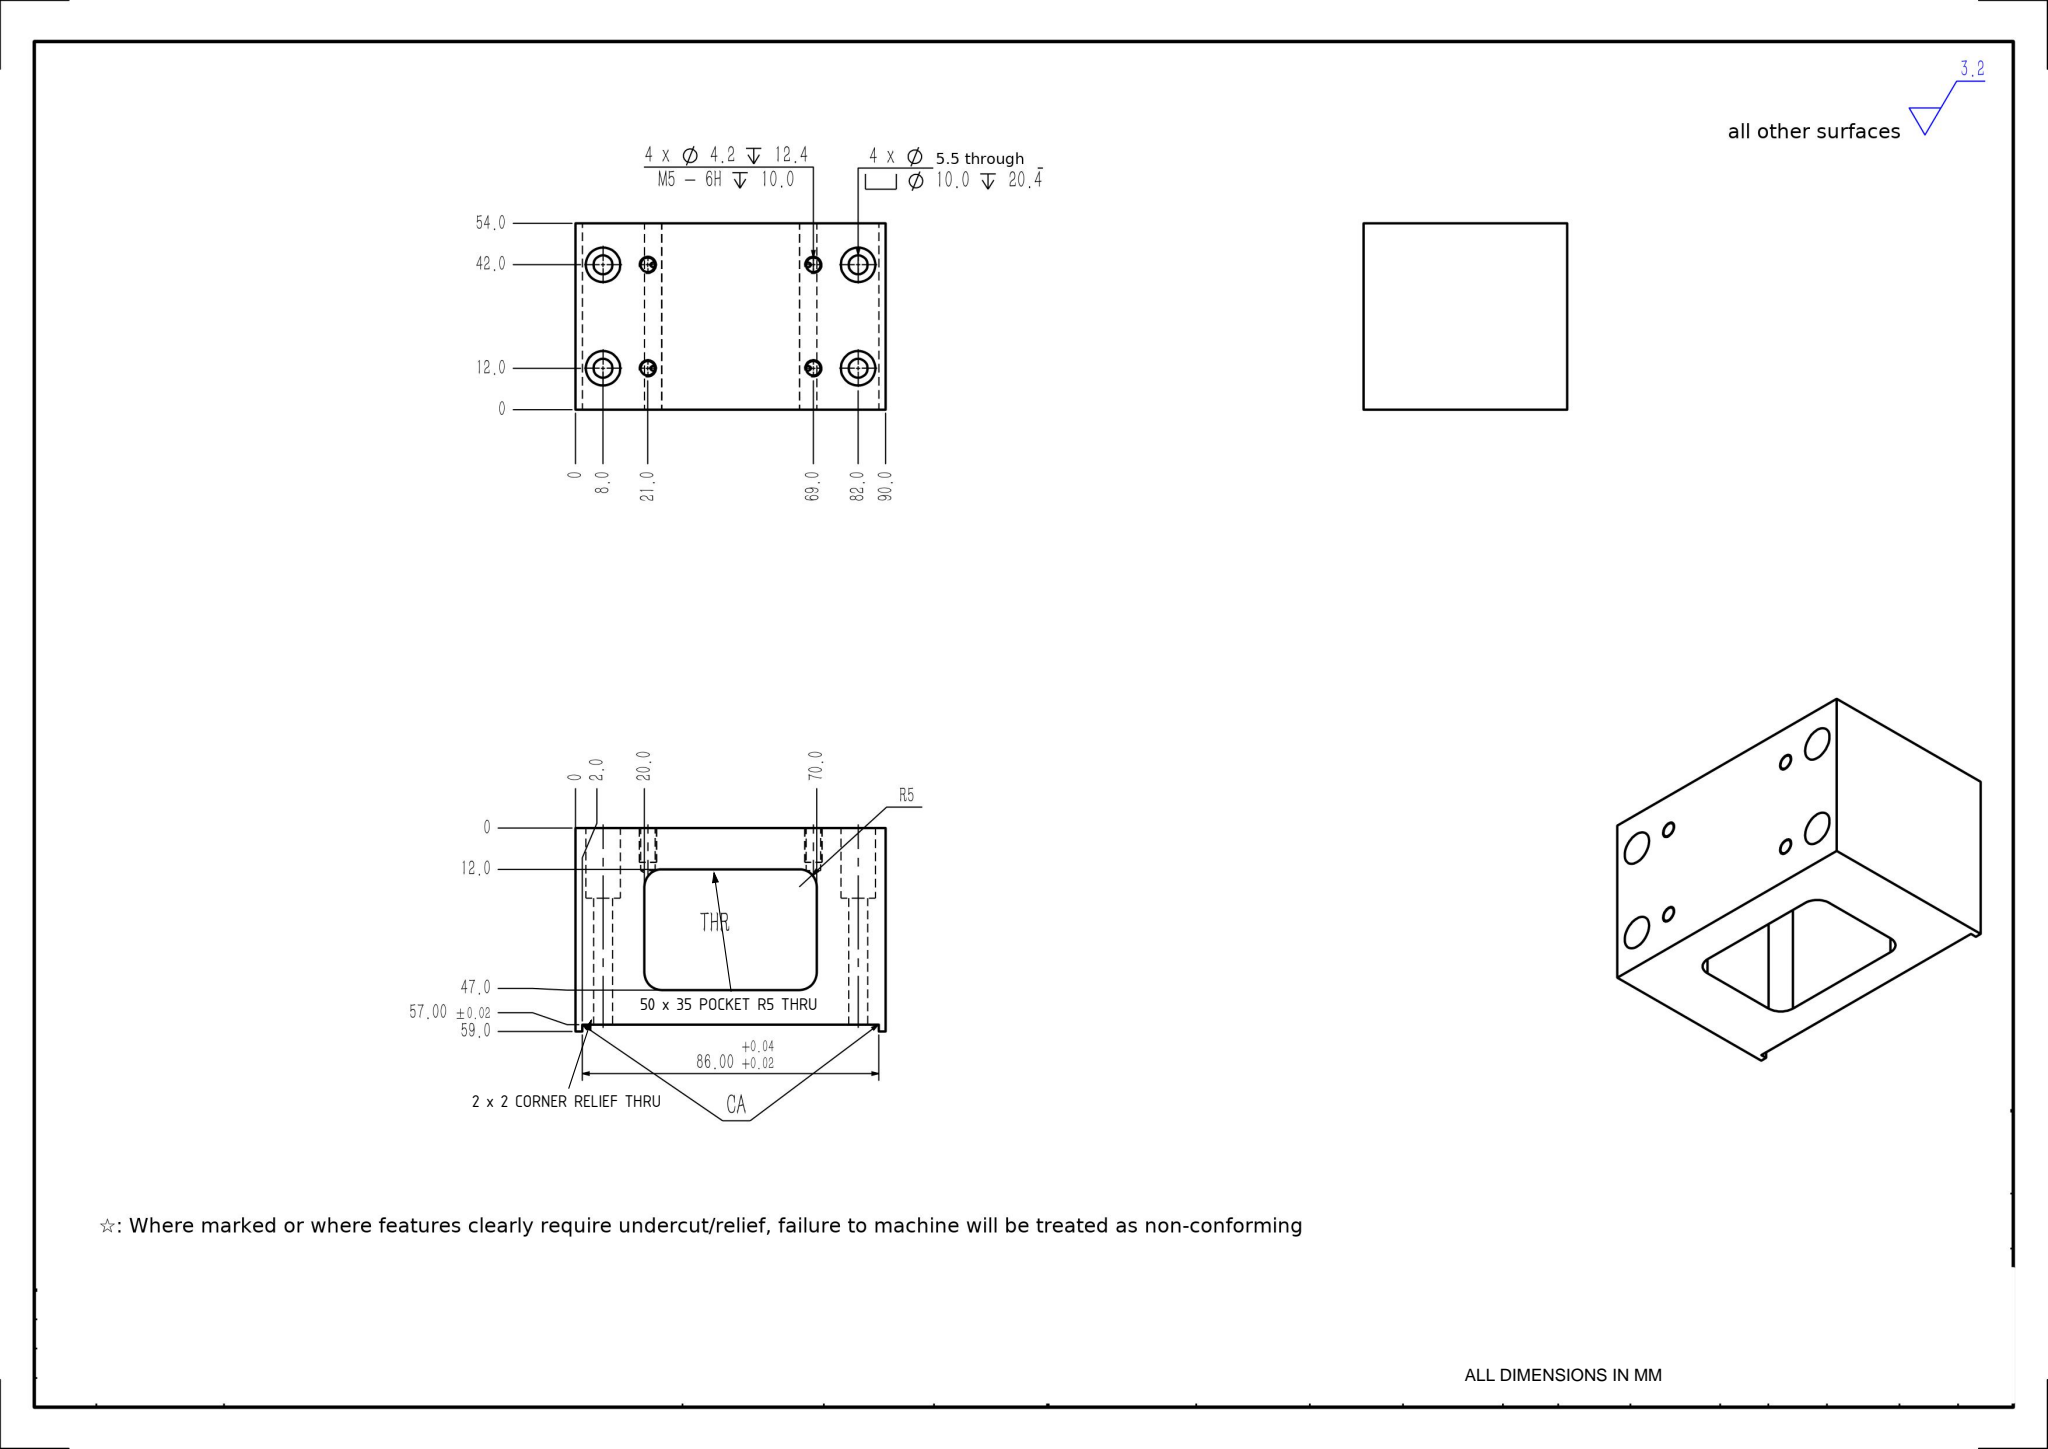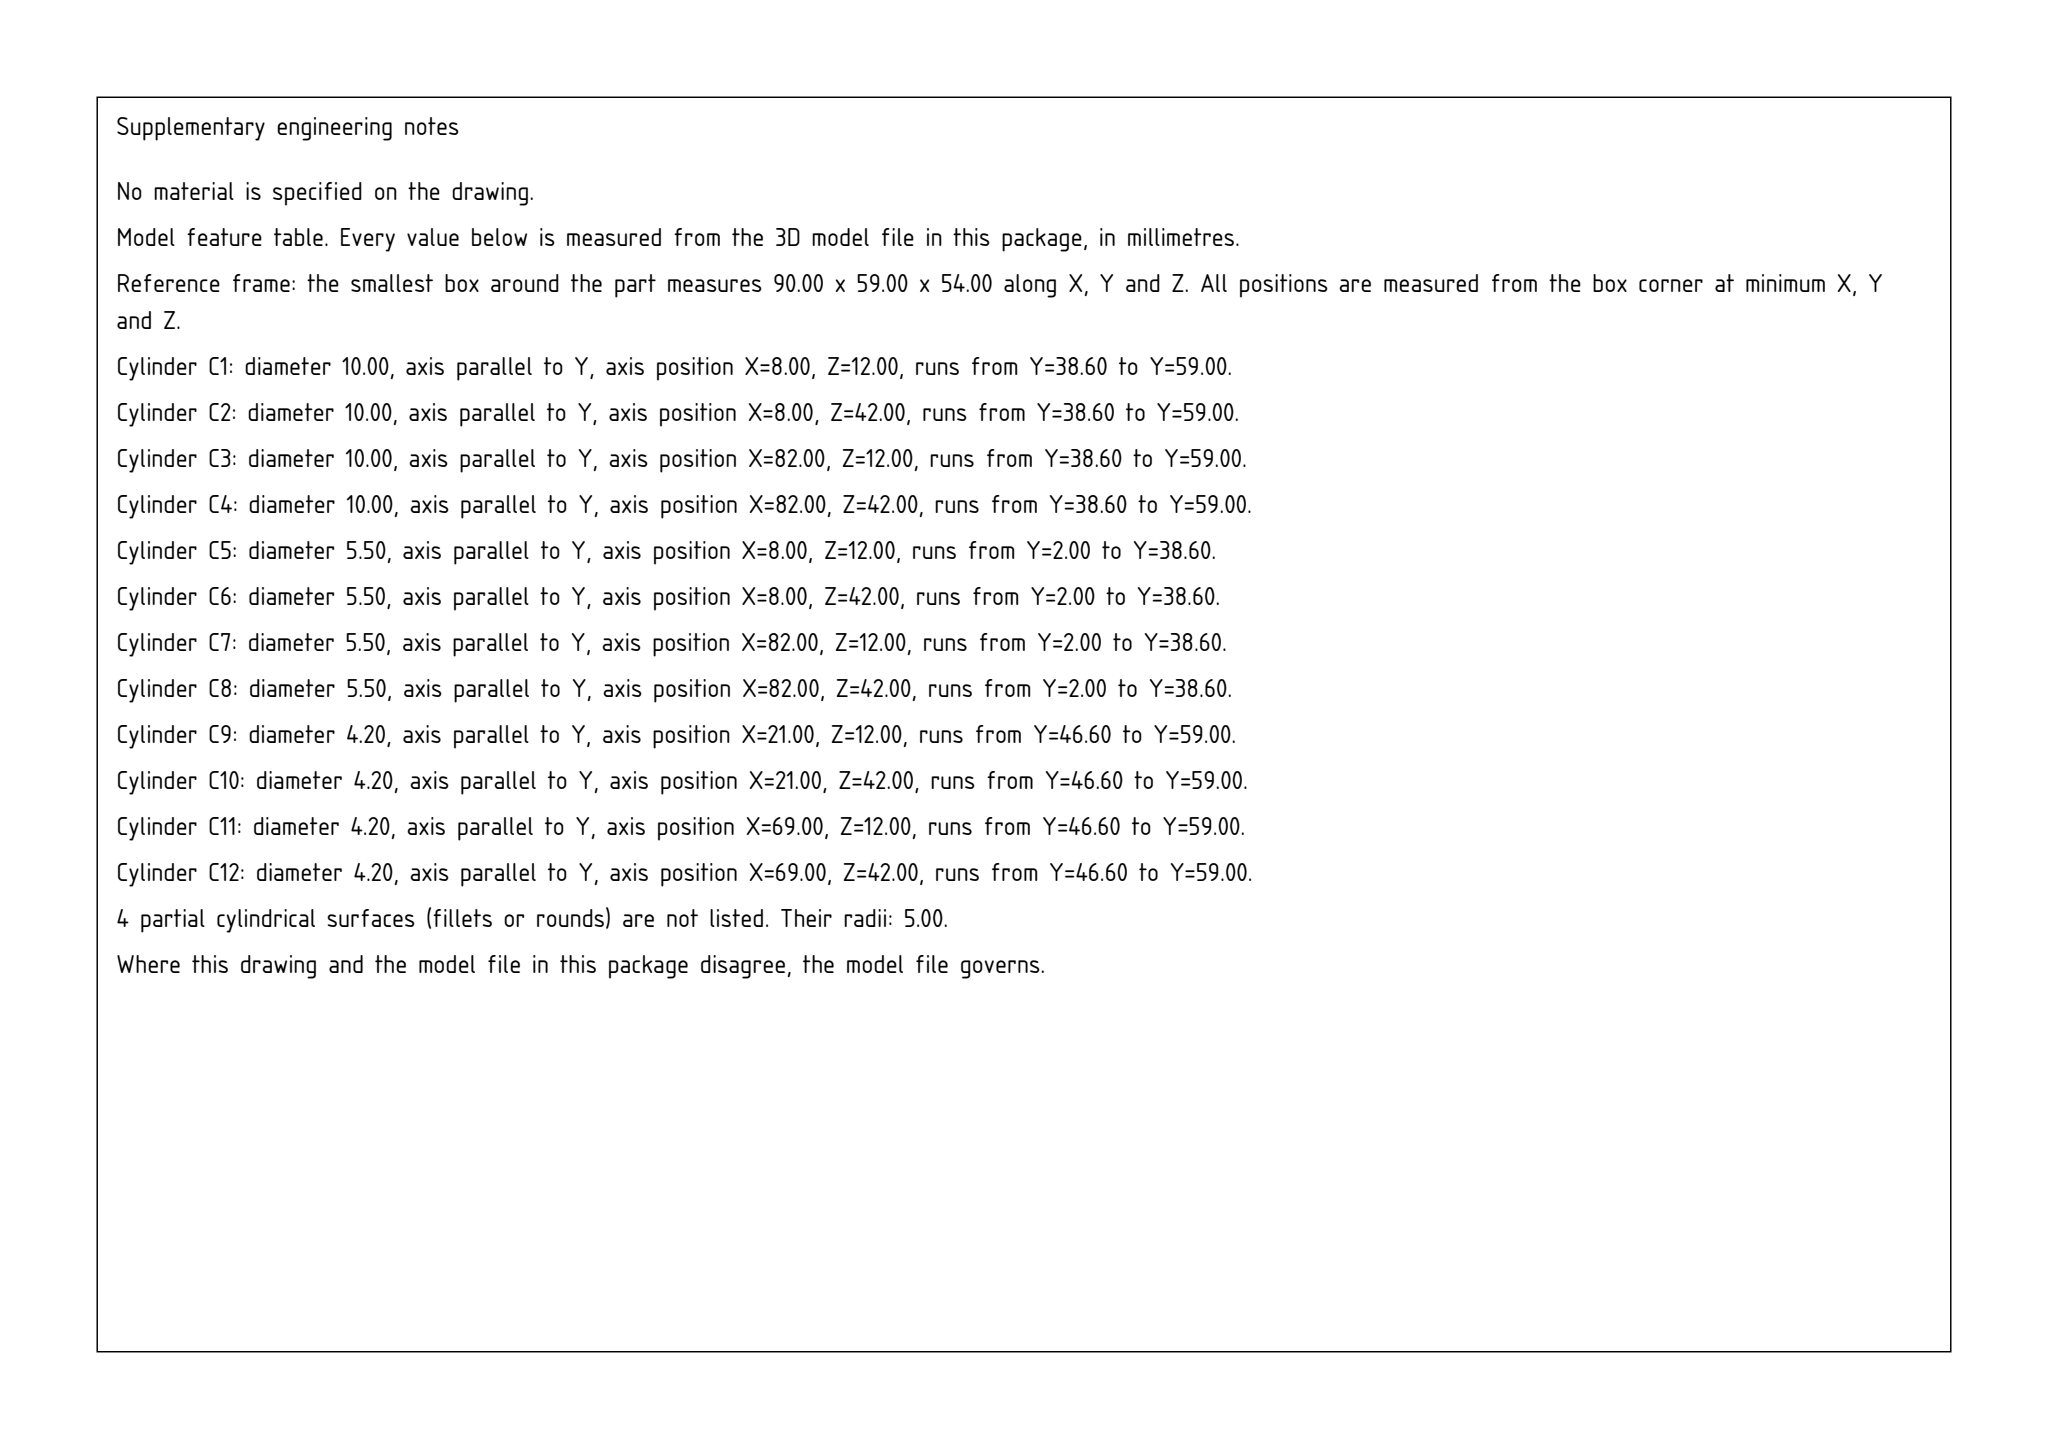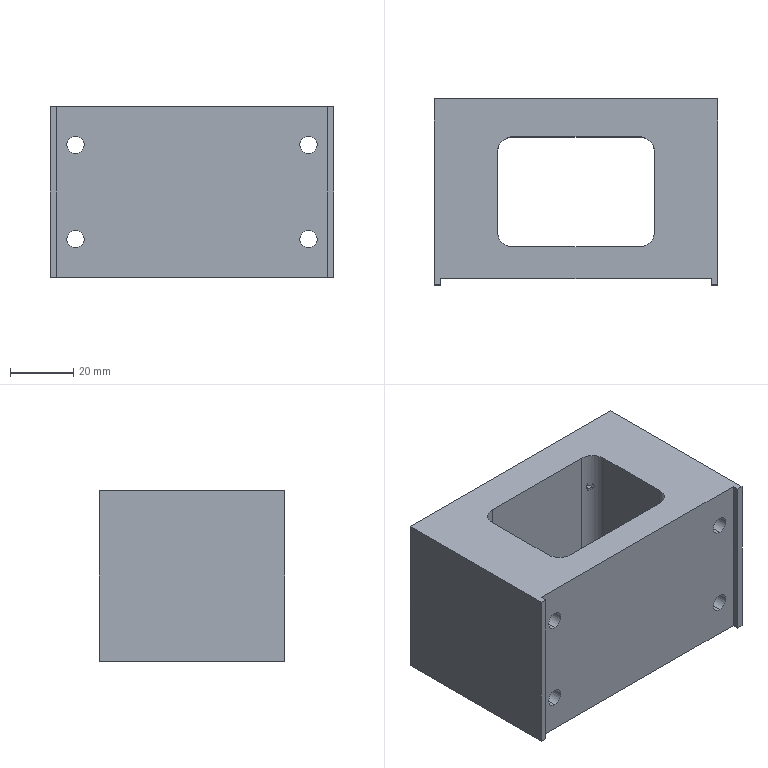Part | SolidWorks | mm | 1 solid | 54 faces | box 90 x 59 x 54 mm | volume 173514 mm3 | cylinder 28 | plane 18 | cone 8 | commonest cylinder face diameters 10 x12 4.2 x8 5.5 x8
Drawing notes:
RECT POCKET 50 x 35, R5 CORNERS, THRU | from the solid: Pocket faces x=20 & x=70 (50 wide), y=12 & y=47 (35 high); four R5 corner cyls Ø10 axis z at (25,17),(25,42),(65,17),(65,42) length 54 = full block depth, i.e. thru
CORNER RELIEF 2 x 2, BOTH BOT CORNERS, THRU 54 DEPTH | from the solid: Planes x=2.0 & x=88.0 (86.00 across) with plane y=2.0 (57.00 from top face y=59) vs bbox 90 x 59 x 54; relief runs full 54 depth
build123d program:
from build123d import *

# Parameters (mm, degrees)
BOSS_EXTRUDE1_DEPTH                             = 27
CUT_EXTRUDE1_DEPTH                              = 77.232
M5_HEX_SOCKET_HEAD_CAP_SCREW_CBORE1_D           = 5.5
M5_HEX_SOCKET_HEAD_CAP_SCREW_CBORE1_CBORE_D     = 10
M5_HEX_SOCKET_HEAD_CAP_SCREW_CBORE1_CBORE_DEPTH = 20.4
M5_TAPPED_HOLE1_D                               = 4.2
M5_TAPPED_HOLE1_DEPTH                           = 12.4
M5_TAPPED_HOLE1_TIP                             = 1.262


with BuildPart() as part:
    # Sketch1 → Boss-Extrude1 (new, symmetric)
    with BuildSketch(Plane.XY):
        Polygon((-43, -29.5), (-43, -27.5), (43, -27.5), (43, -29.5), (45, -29.5), (45, 29.5), (-45, 29.5), (-45, -29.5), align=None)
    extrude(amount=BOSS_EXTRUDE1_DEPTH, both=True)

    # Sketch2 → Cut-Extrude1 (cut, through all)
    with BuildSketch(Plane.XY.offset(27)):
        with BuildLine():
            Line((-20, -17.5), (20, -17.5))
            ThreePointArc((20, -17.5), (23.536, -16.036), (25, -12.5))
            Line((25, -12.5), (25, 12.5))
            ThreePointArc((25, 12.5), (23.536, 16.036), (20, 17.5))
            Line((20, 17.5), (-20, 17.5))
            ThreePointArc((-20, 17.5), (-23.536, 16.036), (-25, 12.5))
            Line((-25, 12.5), (-25, -12.5))
            ThreePointArc((-25, -12.5), (-23.536, -16.036), (-20, -17.5))
        make_face()
    extrude(amount=-CUT_EXTRUDE1_DEPTH, mode=Mode.SUBTRACT)

    # M5 Hex Socket Head Cap Screw CBORE1 (through all)
    with Locations(Plane(origin=(0, 29.5, 0), x_dir=(1, 0, 0), z_dir=(0, 1, 0))):
        with Locations((-37, 15), (-37, -15), (37, 15), (37, -15)):
            CounterBoreHole(M5_HEX_SOCKET_HEAD_CAP_SCREW_CBORE1_D / 2, M5_HEX_SOCKET_HEAD_CAP_SCREW_CBORE1_CBORE_D / 2, M5_HEX_SOCKET_HEAD_CAP_SCREW_CBORE1_CBORE_DEPTH)

    # M5 Tapped Hole1
    with Locations(Plane(origin=(0, 29.5, 0), x_dir=(1, 0, 0), z_dir=(0, 1, 0))):
        with Locations((-24, 15), (24, 15), (-24, -15), (24, -15)):
            Hole(M5_TAPPED_HOLE1_D / 2, depth=M5_TAPPED_HOLE1_DEPTH)
            with Locations((0, 0, -(M5_TAPPED_HOLE1_DEPTH + M5_TAPPED_HOLE1_TIP / 2))):  # 118° drill point
                Cone(0, M5_TAPPED_HOLE1_D / 2, M5_TAPPED_HOLE1_TIP, mode=Mode.SUBTRACT)


solid = part.part